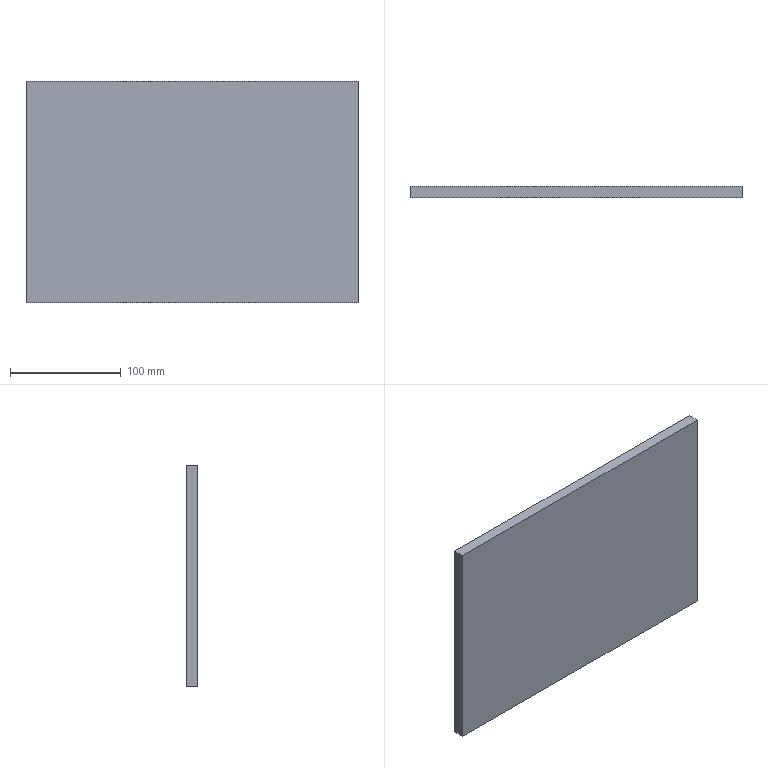Component | NX | F1_2 | 1 solid | 6 faces | box 300 x 10 x 200 mm | volume 600000 mm3 | plane 6
STEP:
#1=CARTESIAN_POINT('',(0.,0.,0.));
#2=DIRECTION('',(0.,0.,1.));
#3=DIRECTION('',(1.,0.,0.));
#4=AXIS2_PLACEMENT_3D('',#1,#2,#3);
#5=CARTESIAN_POINT('',(6480.,-266.,16008.));
#6=VERTEX_POINT('',#5);
#7=CARTESIAN_POINT('',(6180.,-266.,16008.));
#8=VERTEX_POINT('',#7);
#9=CARTESIAN_POINT('',(6480.,-266.,16008.));
#10=DIRECTION('',(-1.,0.,0.));
#11=VECTOR('',#10,1.);
#12=LINE('',#9,#11);
#13=CARTESIAN_POINT('',(6480.,-256.,16008.));
#14=DIRECTION('',(0.,0.,1.));
#15=DIRECTION('',(0.,1.,0.));
#16=AXIS2_PLACEMENT_3D('',#13,#14,#15);
#17=PLANE('',#16);
#18=CARTESIAN_POINT('',(-10.,0.));
#19=DIRECTION('',(0.,1.));
#20=VECTOR('',#19,1.);
#21=LINE('',#18,#20);
#22=(GEOMETRIC_REPRESENTATION_CONTEXT(2)PARAMETRIC_REPRESENTATION_CONTEXT()REPRESENTATION_CONTEXT('',''));
#23=DEFINITIONAL_REPRESENTATION('',(#21),#22);
#24=PCURVE('',#17,#23);
#25=CARTESIAN_POINT('',(6480.,-266.,16008.));
#26=DIRECTION('',(0.,1.,0.));
#27=DIRECTION('',(0.,0.,-1.));
#28=AXIS2_PLACEMENT_3D('',#25,#26,#27);
#29=PLANE('',#28);
#30=CARTESIAN_POINT('',(0.,0.));
#31=DIRECTION('',(0.,1.));
#32=VECTOR('',#31,1.);
#33=LINE('',#30,#32);
#34=(GEOMETRIC_REPRESENTATION_CONTEXT(2)PARAMETRIC_REPRESENTATION_CONTEXT()REPRESENTATION_CONTEXT('',''));
#35=DEFINITIONAL_REPRESENTATION('',(#33),#34);
#36=PCURVE('',#29,#35);
#37=SURFACE_CURVE('',#12,(#24,#36),.PCURVE_S1.);
#38=EDGE_CURVE('',#6,#8,#37,.T.);
#39=ORIENTED_EDGE('',*,*,#38,.T.);
#40=CARTESIAN_POINT('',(6180.,-256.,16008.));
#41=VERTEX_POINT('',#40);
#42=CARTESIAN_POINT('',(6180.,-256.,16008.));
#43=DIRECTION('',(0.,-1.,0.));
#44=VECTOR('',#43,1.);
#45=LINE('',#42,#44);
#46=CARTESIAN_POINT('',(0.,300.));
#47=DIRECTION('',(-1.,0.));
#48=VECTOR('',#47,1.);
#49=LINE('',#46,#48);
#50=(GEOMETRIC_REPRESENTATION_CONTEXT(2)PARAMETRIC_REPRESENTATION_CONTEXT()REPRESENTATION_CONTEXT('',''));
#51=DEFINITIONAL_REPRESENTATION('',(#49),#50);
#52=PCURVE('',#17,#51);
#53=CARTESIAN_POINT('',(6180.,-256.,16008.));
#54=DIRECTION('',(1.,0.,0.));
#55=DIRECTION('',(0.,1.,0.));
#56=AXIS2_PLACEMENT_3D('',#53,#54,#55);
#57=PLANE('',#56);
#58=CARTESIAN_POINT('',(0.,0.));
#59=DIRECTION('',(-1.,0.));
#60=VECTOR('',#59,1.);
#61=LINE('',#58,#60);
#62=(GEOMETRIC_REPRESENTATION_CONTEXT(2)PARAMETRIC_REPRESENTATION_CONTEXT()REPRESENTATION_CONTEXT('',''));
#63=DEFINITIONAL_REPRESENTATION('',(#61),#62);
#64=PCURVE('',#57,#63);
#65=SURFACE_CURVE('',#45,(#52,#64),.PCURVE_S1.);
#66=EDGE_CURVE('',#41,#8,#65,.T.);
#67=ORIENTED_EDGE('',*,*,#66,.F.);
#68=CARTESIAN_POINT('',(6480.,-256.,16008.));
#69=VERTEX_POINT('',#68);
#70=CARTESIAN_POINT('',(6480.,-256.,16008.));
#71=DIRECTION('',(-1.,0.,0.));
#72=VECTOR('',#71,1.);
#73=LINE('',#70,#72);
#74=CARTESIAN_POINT('',(0.,0.));
#75=DIRECTION('',(0.,1.));
#76=VECTOR('',#75,1.);
#77=LINE('',#74,#76);
#78=(GEOMETRIC_REPRESENTATION_CONTEXT(2)PARAMETRIC_REPRESENTATION_CONTEXT()REPRESENTATION_CONTEXT('',''));
#79=DEFINITIONAL_REPRESENTATION('',(#77),#78);
#80=PCURVE('',#17,#79);
#81=CARTESIAN_POINT('',(6480.,-256.,16008.));
#82=DIRECTION('',(0.,1.,0.));
#83=DIRECTION('',(0.,0.,-1.));
#84=AXIS2_PLACEMENT_3D('',#81,#82,#83);
#85=PLANE('',#84);
#86=CARTESIAN_POINT('',(0.,0.));
#87=DIRECTION('',(0.,1.));
#88=VECTOR('',#87,1.);
#89=LINE('',#86,#88);
#90=(GEOMETRIC_REPRESENTATION_CONTEXT(2)PARAMETRIC_REPRESENTATION_CONTEXT()REPRESENTATION_CONTEXT('',''));
#91=DEFINITIONAL_REPRESENTATION('',(#89),#90);
#92=PCURVE('',#85,#91);
#93=SURFACE_CURVE('',#73,(#80,#92),.PCURVE_S1.);
#94=EDGE_CURVE('',#69,#41,#93,.T.);
#95=ORIENTED_EDGE('',*,*,#94,.F.);
#96=CARTESIAN_POINT('',(6480.,-256.,16008.));
#97=DIRECTION('',(0.,-1.,0.));
#98=VECTOR('',#97,1.);
#99=LINE('',#96,#98);
#100=CARTESIAN_POINT('',(0.,0.));
#101=DIRECTION('',(-1.,0.));
#102=VECTOR('',#101,1.);
#103=LINE('',#100,#102);
#104=(GEOMETRIC_REPRESENTATION_CONTEXT(2)PARAMETRIC_REPRESENTATION_CONTEXT()REPRESENTATION_CONTEXT('',''));
#105=DEFINITIONAL_REPRESENTATION('',(#103),#104);
#106=PCURVE('',#17,#105);
#107=CARTESIAN_POINT('',(6480.,-256.,16208.));
#108=DIRECTION('',(-1.,0.,0.));
#109=DIRECTION('',(0.,-1.,0.));
#110=AXIS2_PLACEMENT_3D('',#107,#108,#109);
#111=PLANE('',#110);
#112=CARTESIAN_POINT('',(0.,-200.));
#113=DIRECTION('',(1.,0.));
#114=VECTOR('',#113,1.);
#115=LINE('',#112,#114);
#116=(GEOMETRIC_REPRESENTATION_CONTEXT(2)PARAMETRIC_REPRESENTATION_CONTEXT()REPRESENTATION_CONTEXT('',''));
#117=DEFINITIONAL_REPRESENTATION('',(#115),#116);
#118=PCURVE('',#111,#117);
#119=SURFACE_CURVE('',#99,(#106,#118),.PCURVE_S1.);
#120=EDGE_CURVE('',#69,#6,#119,.T.);
#121=ORIENTED_EDGE('',*,*,#120,.T.);
#122=EDGE_LOOP('',(#39,#67,#95,#121));
#123=FACE_BOUND('',#122,.T.);
#124=ADVANCED_FACE('',(#123),#17,.F.);
#125=CARTESIAN_POINT('',(6180.,-266.,16208.));
#126=VERTEX_POINT('',#125);
#127=CARTESIAN_POINT('',(6180.,-266.,16008.));
#128=DIRECTION('',(0.,0.,1.));
#129=VECTOR('',#128,1.);
#130=LINE('',#127,#129);
#131=CARTESIAN_POINT('',(-10.,0.));
#132=DIRECTION('',(0.,1.));
#133=VECTOR('',#132,1.);
#134=LINE('',#131,#133);
#135=(GEOMETRIC_REPRESENTATION_CONTEXT(2)PARAMETRIC_REPRESENTATION_CONTEXT()REPRESENTATION_CONTEXT('',''));
#136=DEFINITIONAL_REPRESENTATION('',(#134),#135);
#137=PCURVE('',#57,#136);
#138=CARTESIAN_POINT('',(0.,300.));
#139=DIRECTION('',(-1.,0.));
#140=VECTOR('',#139,1.);
#141=LINE('',#138,#140);
#142=(GEOMETRIC_REPRESENTATION_CONTEXT(2)PARAMETRIC_REPRESENTATION_CONTEXT()REPRESENTATION_CONTEXT('',''));
#143=DEFINITIONAL_REPRESENTATION('',(#141),#142);
#144=PCURVE('',#29,#143);
#145=SURFACE_CURVE('',#130,(#137,#144),.PCURVE_S1.);
#146=EDGE_CURVE('',#8,#126,#145,.T.);
#147=ORIENTED_EDGE('',*,*,#146,.T.);
#148=CARTESIAN_POINT('',(6180.,-256.,16208.));
#149=VERTEX_POINT('',#148);
#150=CARTESIAN_POINT('',(6180.,-256.,16208.));
#151=DIRECTION('',(0.,-1.,0.));
#152=VECTOR('',#151,1.);
#153=LINE('',#150,#152);
#154=CARTESIAN_POINT('',(0.,200.));
#155=DIRECTION('',(-1.,0.));
#156=VECTOR('',#155,1.);
#157=LINE('',#154,#156);
#158=(GEOMETRIC_REPRESENTATION_CONTEXT(2)PARAMETRIC_REPRESENTATION_CONTEXT()REPRESENTATION_CONTEXT('',''));
#159=DEFINITIONAL_REPRESENTATION('',(#157),#158);
#160=PCURVE('',#57,#159);
#161=CARTESIAN_POINT('',(6180.,-256.,16208.));
#162=DIRECTION('',(0.,0.,-1.));
#163=DIRECTION('',(0.,-1.,0.));
#164=AXIS2_PLACEMENT_3D('',#161,#162,#163);
#165=PLANE('',#164);
#166=CARTESIAN_POINT('',(0.,0.));
#167=DIRECTION('',(1.,0.));
#168=VECTOR('',#167,1.);
#169=LINE('',#166,#168);
#170=(GEOMETRIC_REPRESENTATION_CONTEXT(2)PARAMETRIC_REPRESENTATION_CONTEXT()REPRESENTATION_CONTEXT('',''));
#171=DEFINITIONAL_REPRESENTATION('',(#169),#170);
#172=PCURVE('',#165,#171);
#173=SURFACE_CURVE('',#153,(#160,#172),.PCURVE_S1.);
#174=EDGE_CURVE('',#149,#126,#173,.T.);
#175=ORIENTED_EDGE('',*,*,#174,.F.);
#176=CARTESIAN_POINT('',(6180.,-256.,16008.));
#177=DIRECTION('',(0.,0.,1.));
#178=VECTOR('',#177,1.);
#179=LINE('',#176,#178);
#180=CARTESIAN_POINT('',(0.,0.));
#181=DIRECTION('',(0.,1.));
#182=VECTOR('',#181,1.);
#183=LINE('',#180,#182);
#184=(GEOMETRIC_REPRESENTATION_CONTEXT(2)PARAMETRIC_REPRESENTATION_CONTEXT()REPRESENTATION_CONTEXT('',''));
#185=DEFINITIONAL_REPRESENTATION('',(#183),#184);
#186=PCURVE('',#57,#185);
#187=CARTESIAN_POINT('',(0.,300.));
#188=DIRECTION('',(-1.,0.));
#189=VECTOR('',#188,1.);
#190=LINE('',#187,#189);
#191=(GEOMETRIC_REPRESENTATION_CONTEXT(2)PARAMETRIC_REPRESENTATION_CONTEXT()REPRESENTATION_CONTEXT('',''));
#192=DEFINITIONAL_REPRESENTATION('',(#190),#191);
#193=PCURVE('',#85,#192);
#194=SURFACE_CURVE('',#179,(#186,#193),.PCURVE_S1.);
#195=EDGE_CURVE('',#41,#149,#194,.T.);
#196=ORIENTED_EDGE('',*,*,#195,.F.);
#197=ORIENTED_EDGE('',*,*,#66,.T.);
#198=EDGE_LOOP('',(#147,#175,#196,#197));
#199=FACE_BOUND('',#198,.T.);
#200=ADVANCED_FACE('',(#199),#57,.F.);
#201=CARTESIAN_POINT('',(6480.,-266.,16208.));
#202=VERTEX_POINT('',#201);
#203=CARTESIAN_POINT('',(6180.,-266.,16208.));
#204=DIRECTION('',(1.,0.,0.));
#205=VECTOR('',#204,1.);
#206=LINE('',#203,#205);
#207=CARTESIAN_POINT('',(10.,0.));
#208=DIRECTION('',(0.,-1.));
#209=VECTOR('',#208,1.);
#210=LINE('',#207,#209);
#211=(GEOMETRIC_REPRESENTATION_CONTEXT(2)PARAMETRIC_REPRESENTATION_CONTEXT()REPRESENTATION_CONTEXT('',''));
#212=DEFINITIONAL_REPRESENTATION('',(#210),#211);
#213=PCURVE('',#165,#212);
#214=CARTESIAN_POINT('',(-200.,300.));
#215=DIRECTION('',(0.,-1.));
#216=VECTOR('',#215,1.);
#217=LINE('',#214,#216);
#218=(GEOMETRIC_REPRESENTATION_CONTEXT(2)PARAMETRIC_REPRESENTATION_CONTEXT()REPRESENTATION_CONTEXT('',''));
#219=DEFINITIONAL_REPRESENTATION('',(#217),#218);
#220=PCURVE('',#29,#219);
#221=SURFACE_CURVE('',#206,(#213,#220),.PCURVE_S1.);
#222=EDGE_CURVE('',#126,#202,#221,.T.);
#223=ORIENTED_EDGE('',*,*,#222,.T.);
#224=CARTESIAN_POINT('',(6480.,-256.,16208.));
#225=VERTEX_POINT('',#224);
#226=CARTESIAN_POINT('',(6480.,-256.,16208.));
#227=DIRECTION('',(0.,-1.,0.));
#228=VECTOR('',#227,1.);
#229=LINE('',#226,#228);
#230=CARTESIAN_POINT('',(0.,-300.));
#231=DIRECTION('',(1.,0.));
#232=VECTOR('',#231,1.);
#233=LINE('',#230,#232);
#234=(GEOMETRIC_REPRESENTATION_CONTEXT(2)PARAMETRIC_REPRESENTATION_CONTEXT()REPRESENTATION_CONTEXT('',''));
#235=DEFINITIONAL_REPRESENTATION('',(#233),#234);
#236=PCURVE('',#165,#235);
#237=CARTESIAN_POINT('',(0.,0.));
#238=DIRECTION('',(1.,0.));
#239=VECTOR('',#238,1.);
#240=LINE('',#237,#239);
#241=(GEOMETRIC_REPRESENTATION_CONTEXT(2)PARAMETRIC_REPRESENTATION_CONTEXT()REPRESENTATION_CONTEXT('',''));
#242=DEFINITIONAL_REPRESENTATION('',(#240),#241);
#243=PCURVE('',#111,#242);
#244=SURFACE_CURVE('',#229,(#236,#243),.PCURVE_S1.);
#245=EDGE_CURVE('',#225,#202,#244,.T.);
#246=ORIENTED_EDGE('',*,*,#245,.F.);
#247=CARTESIAN_POINT('',(6180.,-256.,16208.));
#248=DIRECTION('',(1.,0.,0.));
#249=VECTOR('',#248,1.);
#250=LINE('',#247,#249);
#251=CARTESIAN_POINT('',(0.,0.));
#252=DIRECTION('',(0.,-1.));
#253=VECTOR('',#252,1.);
#254=LINE('',#251,#253);
#255=(GEOMETRIC_REPRESENTATION_CONTEXT(2)PARAMETRIC_REPRESENTATION_CONTEXT()REPRESENTATION_CONTEXT('',''));
#256=DEFINITIONAL_REPRESENTATION('',(#254),#255);
#257=PCURVE('',#165,#256);
#258=CARTESIAN_POINT('',(-200.,300.));
#259=DIRECTION('',(0.,-1.));
#260=VECTOR('',#259,1.);
#261=LINE('',#258,#260);
#262=(GEOMETRIC_REPRESENTATION_CONTEXT(2)PARAMETRIC_REPRESENTATION_CONTEXT()REPRESENTATION_CONTEXT('',''));
#263=DEFINITIONAL_REPRESENTATION('',(#261),#262);
#264=PCURVE('',#85,#263);
#265=SURFACE_CURVE('',#250,(#257,#264),.PCURVE_S1.);
#266=EDGE_CURVE('',#149,#225,#265,.T.);
#267=ORIENTED_EDGE('',*,*,#266,.F.);
#268=ORIENTED_EDGE('',*,*,#174,.T.);
#269=EDGE_LOOP('',(#223,#246,#267,#268));
#270=FACE_BOUND('',#269,.T.);
#271=ADVANCED_FACE('',(#270),#165,.F.);
#272=CARTESIAN_POINT('',(6480.,-266.,16208.));
#273=DIRECTION('',(0.,0.,-1.));
#274=VECTOR('',#273,1.);
#275=LINE('',#272,#274);
#276=CARTESIAN_POINT('',(10.,0.));
#277=DIRECTION('',(0.,-1.));
#278=VECTOR('',#277,1.);
#279=LINE('',#276,#278);
#280=(GEOMETRIC_REPRESENTATION_CONTEXT(2)PARAMETRIC_REPRESENTATION_CONTEXT()REPRESENTATION_CONTEXT('',''));
#281=DEFINITIONAL_REPRESENTATION('',(#279),#280);
#282=PCURVE('',#111,#281);
#283=CARTESIAN_POINT('',(-200.,0.));
#284=DIRECTION('',(1.,0.));
#285=VECTOR('',#284,1.);
#286=LINE('',#283,#285);
#287=(GEOMETRIC_REPRESENTATION_CONTEXT(2)PARAMETRIC_REPRESENTATION_CONTEXT()REPRESENTATION_CONTEXT('',''));
#288=DEFINITIONAL_REPRESENTATION('',(#286),#287);
#289=PCURVE('',#29,#288);
#290=SURFACE_CURVE('',#275,(#282,#289),.PCURVE_S1.);
#291=EDGE_CURVE('',#202,#6,#290,.T.);
#292=ORIENTED_EDGE('',*,*,#291,.T.);
#293=ORIENTED_EDGE('',*,*,#120,.F.);
#294=CARTESIAN_POINT('',(6480.,-256.,16208.));
#295=DIRECTION('',(0.,0.,-1.));
#296=VECTOR('',#295,1.);
#297=LINE('',#294,#296);
#298=CARTESIAN_POINT('',(0.,0.));
#299=DIRECTION('',(0.,-1.));
#300=VECTOR('',#299,1.);
#301=LINE('',#298,#300);
#302=(GEOMETRIC_REPRESENTATION_CONTEXT(2)PARAMETRIC_REPRESENTATION_CONTEXT()REPRESENTATION_CONTEXT('',''));
#303=DEFINITIONAL_REPRESENTATION('',(#301),#302);
#304=PCURVE('',#111,#303);
#305=CARTESIAN_POINT('',(-200.,0.));
#306=DIRECTION('',(1.,0.));
#307=VECTOR('',#306,1.);
#308=LINE('',#305,#307);
#309=(GEOMETRIC_REPRESENTATION_CONTEXT(2)PARAMETRIC_REPRESENTATION_CONTEXT()REPRESENTATION_CONTEXT('',''));
#310=DEFINITIONAL_REPRESENTATION('',(#308),#309);
#311=PCURVE('',#85,#310);
#312=SURFACE_CURVE('',#297,(#304,#311),.PCURVE_S1.);
#313=EDGE_CURVE('',#225,#69,#312,.T.);
#314=ORIENTED_EDGE('',*,*,#313,.F.);
#315=ORIENTED_EDGE('',*,*,#245,.T.);
#316=EDGE_LOOP('',(#292,#293,#314,#315));
#317=FACE_BOUND('',#316,.T.);
#318=ADVANCED_FACE('',(#317),#111,.F.);
#319=ORIENTED_EDGE('',*,*,#94,.T.);
#320=ORIENTED_EDGE('',*,*,#195,.T.);
#321=ORIENTED_EDGE('',*,*,#266,.T.);
#322=ORIENTED_EDGE('',*,*,#313,.T.);
#323=EDGE_LOOP('',(#319,#320,#321,#322));
#324=FACE_BOUND('',#323,.T.);
#325=ADVANCED_FACE('',(#324),#85,.T.);
#326=ORIENTED_EDGE('',*,*,#38,.F.);
#327=ORIENTED_EDGE('',*,*,#291,.F.);
#328=ORIENTED_EDGE('',*,*,#222,.F.);
#329=ORIENTED_EDGE('',*,*,#146,.F.);
#330=EDGE_LOOP('',(#326,#327,#328,#329));
#331=FACE_BOUND('',#330,.T.);
#332=ADVANCED_FACE('',(#331),#29,.F.);
#333=CLOSED_SHELL('',(#124,#200,#271,#318,#325,#332));
#334=MANIFOLD_SOLID_BREP('',#333);
#335=(LENGTH_UNIT()NAMED_UNIT(*)SI_UNIT(.MILLI.,.METRE.));
#336=UNCERTAINTY_MEASURE_WITH_UNIT(LENGTH_MEASURE(0.0000001),#335,'','');
#337=(NAMED_UNIT(*)PLANE_ANGLE_UNIT()SI_UNIT($,.RADIAN.));
#338=(NAMED_UNIT(*)SI_UNIT($,.STERADIAN.)SOLID_ANGLE_UNIT());
#339=(GEOMETRIC_REPRESENTATION_CONTEXT(3)GLOBAL_UNCERTAINTY_ASSIGNED_CONTEXT((#336))GLOBAL_UNIT_ASSIGNED_CONTEXT((#335,#337,#338))REPRESENTATION_CONTEXT('',''));
#340=ADVANCED_BREP_SHAPE_REPRESENTATION('',(#4,#334),#339);